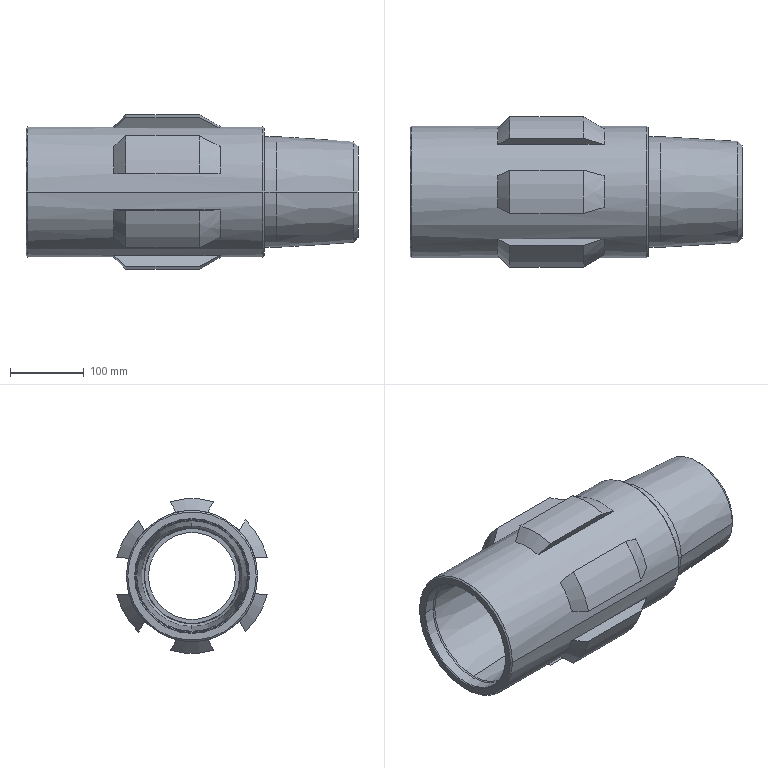Component | SolidWorks | 216OuterTube-1_UpperCentralizer-1 | 1 solid | 67 faces | volume 4982532 mm3 | cone 34 | plane 17 | cylinder 16 | commonest cylinder face diameters 210 x6 130.115 x2 178 x2 150 x2 118 x2 129 x2 | material Alloy Steel